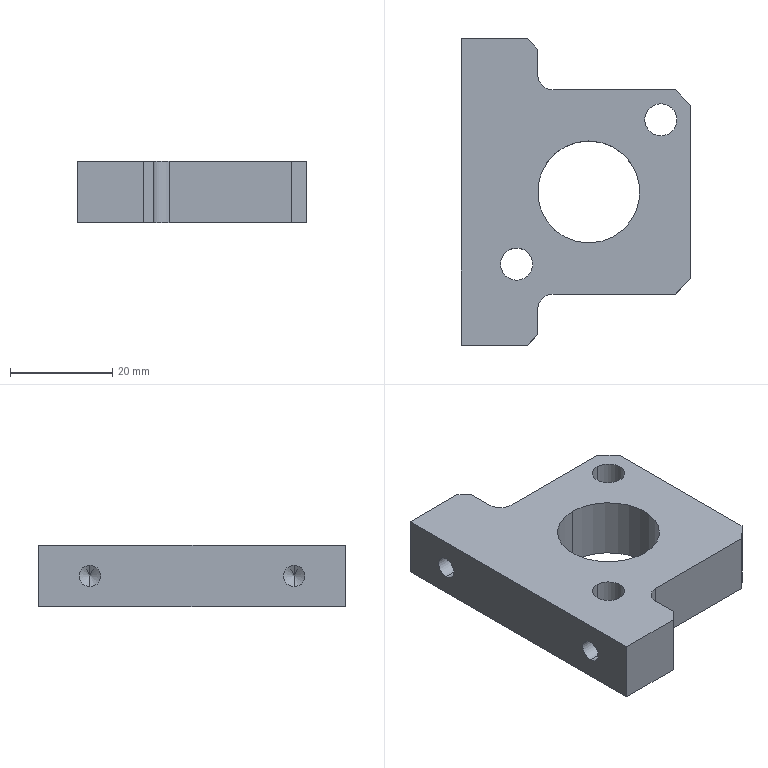Component | SolidWorks | 52-1 | 1 solid | 30 faces | box 45 x 60 x 12 mm | volume 20173 mm3 | plane 14 | cylinder 12 | cone 4 | commonest cylinder face diameters 6.3 x4 4.2 x4 20 x2 6 x2
build123d program:
from build123d import *

# Parameters (mm, degrees)
SKETCH1_R               = 10
BOSS_EXTRUDE1_DEPTH     = 12
FILLET1_R               = 3
M5_TAPPED_HOLE1_D       = 4.2
M5_TAPPED_HOLE1_DEPTH   = 14
M5_TAPPED_HOLE1_TIP     = 1.262
CHAMFER1_SIZE           = 3
SKETCH4_R               = 3.15
CUT_EXTRUDE1_DEPTH      = 12
CIRCULAR_PATTERN1_COUNT = 2
CHAMFER2_SIZE           = 2


with BuildPart() as part:
    # Sketch1 → Boss-Extrude1 (new body)
    with BuildSketch(Plane.XY):
        Polygon((-20, 10), (-30, 10), (-30, 25), (30, 25), (30, 10), (20, 10), (20, -20), (-20, -20), align=None)
        Circle(SKETCH1_R, mode=Mode.SUBTRACT)
    extrude(amount=BOSS_EXTRUDE1_DEPTH)

    # Fillet1
    fillet1_edges = [part.edges().sort_by_distance(p)[0] for p in [
        (20, 10, 6),
        (-20, 10, 6),
    ]]
    fillet(fillet1_edges, radius=FILLET1_R)

    # M5 Tapped Hole1
    with Locations(Plane(origin=(0, 25, 0), x_dir=(1, 0, 0), z_dir=(0, 1, 0))):
        with Locations((-20, -6), (20, -6)):
            Hole(M5_TAPPED_HOLE1_D / 2, depth=M5_TAPPED_HOLE1_DEPTH)
            with Locations((0, 0, -(M5_TAPPED_HOLE1_DEPTH + M5_TAPPED_HOLE1_TIP / 2))):  # 118° drill point
                Cone(0, M5_TAPPED_HOLE1_D / 2, M5_TAPPED_HOLE1_TIP, mode=Mode.SUBTRACT)

    # Chamfer1
    chamfer1_edges = [part.edges().sort_by_distance(p)[0] for p in [
        (20, -20, 6),
        (-20, -20, 6),
    ]]
    chamfer(chamfer1_edges, length=CHAMFER1_SIZE)

    # Sketch4 → Cut-Extrude1 (cut)
    with BuildSketch(Plane.XY.offset(12)):
        with Locations((-14.142, -14.142)):
            Circle(SKETCH4_R)
    cut_extrude1 = extrude(amount=-CUT_EXTRUDE1_DEPTH, mode=Mode.SUBTRACT)

    # Circular Pattern1: Cut-Extrude1 ×2 about axis
    circular_pattern1_axis = Axis((0, 0, 0), (0, 0, 1))
    for i in range(1, CIRCULAR_PATTERN1_COUNT):
        add(cut_extrude1.rotate(circular_pattern1_axis, i * 360 / CIRCULAR_PATTERN1_COUNT), mode=Mode.SUBTRACT)

    # Chamfer2
    chamfer2_edges = [part.edges().sort_by_distance(p)[0] for p in [
        (30, 10, 6),
        (-30, 10, 6),
    ]]
    chamfer(chamfer2_edges, length=CHAMFER2_SIZE)


solid = part.part

# Placed as in the assembly
solid = solid.moved(Location((0, -65.5, 214.893), (180, 0, 90)))
STEP:
#1=CARTESIAN_POINT('',(-0.5568,-3.012,8.46));
#2=VERTEX_POINT('',#1);
#3=CARTESIAN_POINT('',(-0.5568,-3.26,8.46));
#4=VERTEX_POINT('',#3);
#5=CARTESIAN_POINT('',(-0.5568,-3.136,8.46));
#6=DIRECTION('',(0.,-0.,-1.));
#7=DIRECTION('',(0.,1.,0.));
#8=AXIS2_PLACEMENT_3D('',#5,#6,#7);
#9=CIRCLE('',#8,0.124);
#10=EDGE_CURVE('',#2,#4,#9,.T.);
#11=ORIENTED_EDGE('',*,*,#10,.F.);
#12=CARTESIAN_POINT('',(-0.5568,-3.012,7.988));
#13=VERTEX_POINT('',#12);
#14=CARTESIAN_POINT('',(-0.5568,-3.012,8.46));
#15=DIRECTION('',(0.,-0.,-1.));
#16=VECTOR('',#15,39.37);
#17=LINE('',#14,#16);
#18=EDGE_CURVE('',#2,#13,#17,.T.);
#19=ORIENTED_EDGE('',*,*,#18,.T.);
#20=CARTESIAN_POINT('',(-0.5568,-3.26,7.988));
#21=VERTEX_POINT('',#20);
#22=CARTESIAN_POINT('',(-0.5568,-3.136,7.988));
#23=DIRECTION('',(0.,-0.,-1.));
#24=DIRECTION('',(0.,1.,0.));
#25=AXIS2_PLACEMENT_3D('',#22,#23,#24);
#26=CIRCLE('',#25,0.124);
#27=EDGE_CURVE('',#13,#21,#26,.T.);
#28=ORIENTED_EDGE('',*,*,#27,.T.);
#29=CARTESIAN_POINT('',(-0.5568,-3.26,8.46));
#30=DIRECTION('',(0.,-0.,-1.));
#31=VECTOR('',#30,39.37);
#32=LINE('',#29,#31);
#33=EDGE_CURVE('',#4,#21,#32,.T.);
#34=ORIENTED_EDGE('',*,*,#33,.F.);
#35=EDGE_LOOP('',(#11,#19,#28,#34));
#36=FACE_OUTER_BOUND('',#35,.T.);
#37=CARTESIAN_POINT('',(-0.5568,-3.136,8.46));
#38=DIRECTION('',(0.,-0.,-1.));
#39=DIRECTION('',(-0.,-1.,0.));
#40=AXIS2_PLACEMENT_3D('',#37,#38,#39);
#41=CYLINDRICAL_SURFACE('',#40,0.124);
#42=ADVANCED_FACE('',(#36),#41,.F.);
#43=CARTESIAN_POINT('',(0.5568,-1.898,8.46));
#44=VERTEX_POINT('',#43);
#45=CARTESIAN_POINT('',(0.5568,-2.146,8.46));
#46=VERTEX_POINT('',#45);
#47=CARTESIAN_POINT('',(0.5568,-2.022,8.46));
#48=DIRECTION('',(0.,-0.,-1.));
#49=DIRECTION('',(-0.,-1.,0.));
#50=AXIS2_PLACEMENT_3D('',#47,#48,#49);
#51=CIRCLE('',#50,0.124);
#52=EDGE_CURVE('',#44,#46,#51,.T.);
#53=ORIENTED_EDGE('',*,*,#52,.F.);
#54=CARTESIAN_POINT('',(0.5568,-1.898,7.988));
#55=VERTEX_POINT('',#54);
#56=CARTESIAN_POINT('',(0.5568,-1.898,8.46));
#57=DIRECTION('',(0.,-0.,-1.));
#58=VECTOR('',#57,39.37);
#59=LINE('',#56,#58);
#60=EDGE_CURVE('',#44,#55,#59,.T.);
#61=ORIENTED_EDGE('',*,*,#60,.T.);
#62=CARTESIAN_POINT('',(0.5568,-2.146,7.988));
#63=VERTEX_POINT('',#62);
#64=CARTESIAN_POINT('',(0.5568,-2.022,7.988));
#65=DIRECTION('',(0.,-0.,-1.));
#66=DIRECTION('',(-0.,-1.,0.));
#67=AXIS2_PLACEMENT_3D('',#64,#65,#66);
#68=CIRCLE('',#67,0.124);
#69=EDGE_CURVE('',#55,#63,#68,.T.);
#70=ORIENTED_EDGE('',*,*,#69,.T.);
#71=CARTESIAN_POINT('',(0.5568,-2.146,8.46));
#72=DIRECTION('',(0.,-0.,-1.));
#73=VECTOR('',#72,39.37);
#74=LINE('',#71,#73);
#75=EDGE_CURVE('',#46,#63,#74,.T.);
#76=ORIENTED_EDGE('',*,*,#75,.F.);
#77=EDGE_LOOP('',(#53,#61,#70,#76));
#78=FACE_OUTER_BOUND('',#77,.T.);
#79=CARTESIAN_POINT('',(0.5568,-2.022,8.46));
#80=DIRECTION('',(0.,-0.,-1.));
#81=DIRECTION('',(-0.,-1.,0.));
#82=AXIS2_PLACEMENT_3D('',#79,#80,#81);
#83=CYLINDRICAL_SURFACE('',#82,0.124);
#84=ADVANCED_FACE('',(#78),#83,.F.);
#85=CARTESIAN_POINT('',(-0.4331,-1.791,8.307));
#86=VERTEX_POINT('',#85);
#87=CARTESIAN_POINT('',(-0.4331,-1.791,8.141));
#88=VERTEX_POINT('',#87);
#89=CARTESIAN_POINT('',(-0.4331,-1.791,8.224));
#90=DIRECTION('',(-1.,0.,-0.));
#91=DIRECTION('',(0.,0.,-1.));
#92=AXIS2_PLACEMENT_3D('',#89,#90,#91);
#93=CIRCLE('',#92,0.08268);
#94=EDGE_CURVE('',#86,#88,#93,.T.);
#95=ORIENTED_EDGE('',*,*,#94,.F.);
#96=CARTESIAN_POINT('',(-0.9843,-1.791,8.307));
#97=VERTEX_POINT('',#96);
#98=CARTESIAN_POINT('',(-0.9843,-1.791,8.307));
#99=DIRECTION('',(-1.,0.,-0.));
#100=VECTOR('',#99,39.37);
#101=LINE('',#98,#100);
#102=EDGE_CURVE('',#86,#97,#101,.T.);
#103=ORIENTED_EDGE('',*,*,#102,.T.);
#104=CARTESIAN_POINT('',(-0.9843,-1.791,8.141));
#105=VERTEX_POINT('',#104);
#106=CARTESIAN_POINT('',(-0.9843,-1.791,8.224));
#107=DIRECTION('',(-1.,0.,-0.));
#108=DIRECTION('',(0.,0.,-1.));
#109=AXIS2_PLACEMENT_3D('',#106,#107,#108);
#110=CIRCLE('',#109,0.08268);
#111=EDGE_CURVE('',#97,#105,#110,.T.);
#112=ORIENTED_EDGE('',*,*,#111,.T.);
#113=CARTESIAN_POINT('',(-0.9843,-1.791,8.141));
#114=DIRECTION('',(-1.,0.,-0.));
#115=VECTOR('',#114,39.37);
#116=LINE('',#113,#115);
#117=EDGE_CURVE('',#88,#105,#116,.T.);
#118=ORIENTED_EDGE('',*,*,#117,.F.);
#119=EDGE_LOOP('',(#95,#103,#112,#118));
#120=FACE_OUTER_BOUND('',#119,.T.);
#121=CARTESIAN_POINT('',(-0.9843,-1.791,8.224));
#122=DIRECTION('',(-1.,0.,-0.));
#123=DIRECTION('',(0.,0.,-1.));
#124=AXIS2_PLACEMENT_3D('',#121,#122,#123);
#125=CYLINDRICAL_SURFACE('',#124,0.08268);
#126=ADVANCED_FACE('',(#120),#125,.F.);
#127=CARTESIAN_POINT('',(-0.3834,-1.791,8.224));
#128=VERTEX_POINT('',#127);
#129=CARTESIAN_POINT('',(-0.4331,-1.791,8.141));
#130=DIRECTION('',(-0.515,0.,-0.8572));
#131=VECTOR('',#130,39.37);
#132=LINE('',#129,#131);
#133=EDGE_CURVE('',#128,#88,#132,.T.);
#134=ORIENTED_EDGE('',*,*,#133,.F.);
#135=CARTESIAN_POINT('',(-0.4331,-1.791,8.307));
#136=DIRECTION('',(-0.515,0.,0.8572));
#137=VECTOR('',#136,39.37);
#138=LINE('',#135,#137);
#139=EDGE_CURVE('',#128,#86,#138,.T.);
#140=ORIENTED_EDGE('',*,*,#139,.T.);
#141=ORIENTED_EDGE('',*,*,#94,.T.);
#142=EDGE_LOOP('',(#134,#140,#141));
#143=FACE_OUTER_BOUND('',#142,.T.);
#144=CARTESIAN_POINT('',(-0.4331,-1.791,8.224));
#145=DIRECTION('',(-1.,0.,-0.));
#146=DIRECTION('',(0.,0.,-1.));
#147=AXIS2_PLACEMENT_3D('',#144,#145,#146);
#148=CONICAL_SURFACE('',#147,0.08268,1.03);
#149=ADVANCED_FACE('',(#143),#148,.F.);
#150=CARTESIAN_POINT('',(-0.4331,-3.366,8.307));
#151=VERTEX_POINT('',#150);
#152=CARTESIAN_POINT('',(-0.4331,-3.366,8.141));
#153=VERTEX_POINT('',#152);
#154=CARTESIAN_POINT('',(-0.4331,-3.366,8.224));
#155=DIRECTION('',(-1.,0.,-0.));
#156=DIRECTION('',(0.,0.,-1.));
#157=AXIS2_PLACEMENT_3D('',#154,#155,#156);
#158=CIRCLE('',#157,0.08268);
#159=EDGE_CURVE('',#151,#153,#158,.T.);
#160=ORIENTED_EDGE('',*,*,#159,.F.);
#161=CARTESIAN_POINT('',(-0.9843,-3.366,8.307));
#162=VERTEX_POINT('',#161);
#163=CARTESIAN_POINT('',(-0.9843,-3.366,8.307));
#164=DIRECTION('',(-1.,0.,-0.));
#165=VECTOR('',#164,39.37);
#166=LINE('',#163,#165);
#167=EDGE_CURVE('',#151,#162,#166,.T.);
#168=ORIENTED_EDGE('',*,*,#167,.T.);
#169=CARTESIAN_POINT('',(-0.9843,-3.366,8.141));
#170=VERTEX_POINT('',#169);
#171=CARTESIAN_POINT('',(-0.9843,-3.366,8.224));
#172=DIRECTION('',(-1.,0.,-0.));
#173=DIRECTION('',(0.,0.,-1.));
#174=AXIS2_PLACEMENT_3D('',#171,#172,#173);
#175=CIRCLE('',#174,0.08268);
#176=EDGE_CURVE('',#162,#170,#175,.T.);
#177=ORIENTED_EDGE('',*,*,#176,.T.);
#178=CARTESIAN_POINT('',(-0.9843,-3.366,8.141));
#179=DIRECTION('',(-1.,0.,-0.));
#180=VECTOR('',#179,39.37);
#181=LINE('',#178,#180);
#182=EDGE_CURVE('',#153,#170,#181,.T.);
#183=ORIENTED_EDGE('',*,*,#182,.F.);
#184=EDGE_LOOP('',(#160,#168,#177,#183));
#185=FACE_OUTER_BOUND('',#184,.T.);
#186=CARTESIAN_POINT('',(-0.9843,-3.366,8.224));
#187=DIRECTION('',(-1.,0.,-0.));
#188=DIRECTION('',(0.,0.,-1.));
#189=AXIS2_PLACEMENT_3D('',#186,#187,#188);
#190=CYLINDRICAL_SURFACE('',#189,0.08268);
#191=ADVANCED_FACE('',(#185),#190,.F.);
#192=CARTESIAN_POINT('',(-0.3834,-3.366,8.224));
#193=VERTEX_POINT('',#192);
#194=CARTESIAN_POINT('',(-0.4331,-3.366,8.141));
#195=DIRECTION('',(-0.515,0.,-0.8572));
#196=VECTOR('',#195,39.37);
#197=LINE('',#194,#196);
#198=EDGE_CURVE('',#193,#153,#197,.T.);
#199=ORIENTED_EDGE('',*,*,#198,.F.);
#200=CARTESIAN_POINT('',(-0.4331,-3.366,8.307));
#201=DIRECTION('',(-0.515,0.,0.8572));
#202=VECTOR('',#201,39.37);
#203=LINE('',#200,#202);
#204=EDGE_CURVE('',#193,#151,#203,.T.);
#205=ORIENTED_EDGE('',*,*,#204,.T.);
#206=ORIENTED_EDGE('',*,*,#159,.T.);
#207=EDGE_LOOP('',(#199,#205,#206));
#208=FACE_OUTER_BOUND('',#207,.T.);
#209=CARTESIAN_POINT('',(-0.4331,-3.366,8.224));
#210=DIRECTION('',(-1.,0.,-0.));
#211=DIRECTION('',(0.,0.,-1.));
#212=AXIS2_PLACEMENT_3D('',#209,#210,#211);
#213=CONICAL_SURFACE('',#212,0.08268,1.03);
#214=ADVANCED_FACE('',(#208),#213,.F.);
#215=CARTESIAN_POINT('',(-0.,-2.185,7.988));
#216=VERTEX_POINT('',#215);
#217=CARTESIAN_POINT('',(-0.,-2.972,7.988));
#218=VERTEX_POINT('',#217);
#219=CARTESIAN_POINT('',(-0.,-2.579,7.988));
#220=DIRECTION('',(0.,-0.,-1.));
#221=DIRECTION('',(-0.,-1.,0.));
#222=AXIS2_PLACEMENT_3D('',#219,#220,#221);
#223=CIRCLE('',#222,0.3937);
#224=EDGE_CURVE('',#216,#218,#223,.T.);
#225=ORIENTED_EDGE('',*,*,#224,.T.);
#226=CARTESIAN_POINT('',(-0.,-2.972,8.46));
#227=VERTEX_POINT('',#226);
#228=CARTESIAN_POINT('',(-0.,-2.972,7.988));
#229=DIRECTION('',(-0.,0.,1.));
#230=VECTOR('',#229,39.37);
#231=LINE('',#228,#230);
#232=EDGE_CURVE('',#218,#227,#231,.T.);
#233=ORIENTED_EDGE('',*,*,#232,.T.);
#234=CARTESIAN_POINT('',(-0.,-2.185,8.46));
#235=VERTEX_POINT('',#234);
#236=CARTESIAN_POINT('',(-0.,-2.579,8.46));
#237=DIRECTION('',(0.,-0.,-1.));
#238=DIRECTION('',(-0.,-1.,0.));
#239=AXIS2_PLACEMENT_3D('',#236,#237,#238);
#240=CIRCLE('',#239,0.3937);
#241=EDGE_CURVE('',#235,#227,#240,.T.);
#242=ORIENTED_EDGE('',*,*,#241,.F.);
#243=CARTESIAN_POINT('',(-0.,-2.185,7.988));
#244=DIRECTION('',(-0.,0.,1.));
#245=VECTOR('',#244,39.37);
#246=LINE('',#243,#245);
#247=EDGE_CURVE('',#216,#235,#246,.T.);
#248=ORIENTED_EDGE('',*,*,#247,.F.);
#249=EDGE_LOOP('',(#225,#233,#242,#248));
#250=FACE_OUTER_BOUND('',#249,.T.);
#251=CARTESIAN_POINT('',(-0.,-2.579,7.988));
#252=DIRECTION('',(-0.,0.,1.));
#253=DIRECTION('',(0.,1.,0.));
#254=AXIS2_PLACEMENT_3D('',#251,#252,#253);
#255=CYLINDRICAL_SURFACE('',#254,0.3937);
#256=ADVANCED_FACE('',(#250),#255,.F.);
#257=CARTESIAN_POINT('',(-0.5568,-3.136,7.988));
#258=DIRECTION('',(0.,-0.,-1.));
#259=DIRECTION('',(0.,1.,0.));
#260=AXIS2_PLACEMENT_3D('',#257,#258,#259);
#261=CIRCLE('',#260,0.124);
#262=EDGE_CURVE('',#21,#13,#261,.T.);
#263=ORIENTED_EDGE('',*,*,#262,.F.);
#264=ORIENTED_EDGE('',*,*,#27,.F.);
#265=EDGE_LOOP('',(#263,#264));
#266=FACE_BOUND('',#265,.T.);
#267=CARTESIAN_POINT('',(0.5568,-2.022,7.988));
#268=DIRECTION('',(0.,-0.,-1.));
#269=DIRECTION('',(-0.,-1.,0.));
#270=AXIS2_PLACEMENT_3D('',#267,#268,#269);
#271=CIRCLE('',#270,0.124);
#272=EDGE_CURVE('',#63,#55,#271,.T.);
#273=ORIENTED_EDGE('',*,*,#272,.F.);
#274=ORIENTED_EDGE('',*,*,#69,.F.);
#275=EDGE_LOOP('',(#273,#274));
#276=FACE_BOUND('',#275,.T.);
#277=CARTESIAN_POINT('',(-0.3937,-3.484,7.988));
#278=VERTEX_POINT('',#277);
#279=CARTESIAN_POINT('',(-0.3937,-3.681,7.988));
#280=VERTEX_POINT('',#279);
#281=CARTESIAN_POINT('',(-0.3937,-3.366,7.988));
#282=DIRECTION('',(-0.,-1.,0.));
#283=VECTOR('',#282,39.37);
#284=LINE('',#281,#283);
#285=EDGE_CURVE('',#278,#280,#284,.T.);
#286=ORIENTED_EDGE('',*,*,#285,.T.);
#287=CARTESIAN_POINT('',(-0.4724,-3.76,7.988));
#288=VERTEX_POINT('',#287);
#289=CARTESIAN_POINT('',(-0.4724,-3.76,7.988));
#290=DIRECTION('',(-0.7071,-0.7071,0.));
#291=VECTOR('',#290,39.37);
#292=LINE('',#289,#291);
#293=EDGE_CURVE('',#280,#288,#292,.T.);
#294=ORIENTED_EDGE('',*,*,#293,.T.);
#295=CARTESIAN_POINT('',(-0.9843,-3.76,7.988));
#296=VERTEX_POINT('',#295);
#297=CARTESIAN_POINT('',(-0.3937,-3.76,7.988));
#298=DIRECTION('',(-1.,0.,-0.));
#299=VECTOR('',#298,39.37);
#300=LINE('',#297,#299);
#301=EDGE_CURVE('',#288,#296,#300,.T.);
#302=ORIENTED_EDGE('',*,*,#301,.T.);
#303=CARTESIAN_POINT('',(-0.9843,-1.398,7.988));
#304=VERTEX_POINT('',#303);
#305=CARTESIAN_POINT('',(-0.9843,-1.398,7.988));
#306=DIRECTION('',(0.,1.,-0.));
#307=VECTOR('',#306,39.37);
#308=LINE('',#305,#307);
#309=EDGE_CURVE('',#296,#304,#308,.T.);
#310=ORIENTED_EDGE('',*,*,#309,.T.);
#311=CARTESIAN_POINT('',(-0.4724,-1.398,7.988));
#312=VERTEX_POINT('',#311);
#313=CARTESIAN_POINT('',(-0.3937,-1.398,7.988));
#314=DIRECTION('',(1.,-0.,0.));
#315=VECTOR('',#314,39.37);
#316=LINE('',#313,#315);
#317=EDGE_CURVE('',#304,#312,#316,.T.);
#318=ORIENTED_EDGE('',*,*,#317,.T.);
#319=CARTESIAN_POINT('',(-0.3937,-1.476,7.988));
#320=VERTEX_POINT('',#319);
#321=CARTESIAN_POINT('',(-0.3937,-1.476,7.988));
#322=DIRECTION('',(0.7071,-0.7071,0.));
#323=VECTOR('',#322,39.37);
#324=LINE('',#321,#323);
#325=EDGE_CURVE('',#312,#320,#324,.T.);
#326=ORIENTED_EDGE('',*,*,#325,.T.);
#327=CARTESIAN_POINT('',(-0.3937,-1.673,7.988));
#328=VERTEX_POINT('',#327);
#329=CARTESIAN_POINT('',(-0.3937,-1.791,7.988));
#330=DIRECTION('',(-0.,-1.,0.));
#331=VECTOR('',#330,39.37);
#332=LINE('',#329,#331);
#333=EDGE_CURVE('',#320,#328,#332,.T.);
#334=ORIENTED_EDGE('',*,*,#333,.T.);
#335=CARTESIAN_POINT('',(-0.2756,-1.791,7.988));
#336=VERTEX_POINT('',#335);
#337=CARTESIAN_POINT('',(-0.2756,-1.673,7.988));
#338=DIRECTION('',(-0.,0.,1.));
#339=DIRECTION('',(0.,1.,0.));
#340=AXIS2_PLACEMENT_3D('',#337,#338,#339);
#341=CIRCLE('',#340,0.1181);
#342=EDGE_CURVE('',#328,#336,#341,.T.);
#343=ORIENTED_EDGE('',*,*,#342,.T.);
#344=CARTESIAN_POINT('',(0.6693,-1.791,7.988));
#345=VERTEX_POINT('',#344);
#346=CARTESIAN_POINT('',(-0.3937,-1.791,7.988));
#347=DIRECTION('',(1.,-0.,0.));
#348=VECTOR('',#347,39.37);
#349=LINE('',#346,#348);
#350=EDGE_CURVE('',#336,#345,#349,.T.);
#351=ORIENTED_EDGE('',*,*,#350,.T.);
#352=CARTESIAN_POINT('',(0.7874,-1.909,7.988));
#353=VERTEX_POINT('',#352);
#354=CARTESIAN_POINT('',(0.7874,-1.909,7.988));
#355=DIRECTION('',(0.7071,-0.7071,0.));
#356=VECTOR('',#355,39.37);
#357=LINE('',#354,#356);
#358=EDGE_CURVE('',#345,#353,#357,.T.);
#359=ORIENTED_EDGE('',*,*,#358,.T.);
#360=CARTESIAN_POINT('',(0.7874,-3.248,7.988));
#361=VERTEX_POINT('',#360);
#362=CARTESIAN_POINT('',(0.7874,-1.791,7.988));
#363=DIRECTION('',(-0.,-1.,0.));
#364=VECTOR('',#363,39.37);
#365=LINE('',#362,#364);
#366=EDGE_CURVE('',#353,#361,#365,.T.);
#367=ORIENTED_EDGE('',*,*,#366,.T.);
#368=CARTESIAN_POINT('',(0.6693,-3.366,7.988));
#369=VERTEX_POINT('',#368);
#370=CARTESIAN_POINT('',(0.6693,-3.366,7.988));
#371=DIRECTION('',(-0.7071,-0.7071,0.));
#372=VECTOR('',#371,39.37);
#373=LINE('',#370,#372);
#374=EDGE_CURVE('',#361,#369,#373,.T.);
#375=ORIENTED_EDGE('',*,*,#374,.T.);
#376=CARTESIAN_POINT('',(-0.2756,-3.366,7.988));
#377=VERTEX_POINT('',#376);
#378=CARTESIAN_POINT('',(-0.3937,-3.366,7.988));
#379=DIRECTION('',(-1.,0.,-0.));
#380=VECTOR('',#379,39.37);
#381=LINE('',#378,#380);
#382=EDGE_CURVE('',#369,#377,#381,.T.);
#383=ORIENTED_EDGE('',*,*,#382,.T.);
#384=CARTESIAN_POINT('',(-0.2756,-3.484,7.988));
#385=DIRECTION('',(-0.,0.,1.));
#386=DIRECTION('',(0.,1.,0.));
#387=AXIS2_PLACEMENT_3D('',#384,#385,#386);
#388=CIRCLE('',#387,0.1181);
#389=EDGE_CURVE('',#377,#278,#388,.T.);
#390=ORIENTED_EDGE('',*,*,#389,.T.);
#391=EDGE_LOOP('',(#286,#294,#302,#310,#318,#326,#334,#343,#351,#359,#367,#375,#383,#390));
#392=FACE_OUTER_BOUND('',#391,.T.);
#393=ORIENTED_EDGE('',*,*,#224,.F.);
#394=CARTESIAN_POINT('',(-0.,-2.579,7.988));
#395=DIRECTION('',(0.,-0.,-1.));
#396=DIRECTION('',(-0.,-1.,0.));
#397=AXIS2_PLACEMENT_3D('',#394,#395,#396);
#398=CIRCLE('',#397,0.3937);
#399=EDGE_CURVE('',#218,#216,#398,.T.);
#400=ORIENTED_EDGE('',*,*,#399,.F.);
#401=EDGE_LOOP('',(#393,#400));
#402=FACE_BOUND('',#401,.T.);
#403=CARTESIAN_POINT('',(-0.,-2.579,7.988));
#404=DIRECTION('',(-0.,0.,1.));
#405=DIRECTION('',(0.,1.,-0.));
#406=AXIS2_PLACEMENT_3D('',#403,#404,#405);
#407=PLANE('',#406);
#408=ADVANCED_FACE('',(#266,#276,#392,#402),#407,.F.);
#409=CARTESIAN_POINT('',(-0.5568,-3.136,8.46));
#410=DIRECTION('',(0.,-0.,-1.));
#411=DIRECTION('',(0.,1.,0.));
#412=AXIS2_PLACEMENT_3D('',#409,#410,#411);
#413=CIRCLE('',#412,0.124);
#414=EDGE_CURVE('',#4,#2,#413,.T.);
#415=ORIENTED_EDGE('',*,*,#414,.T.);
#416=ORIENTED_EDGE('',*,*,#10,.T.);
#417=EDGE_LOOP('',(#415,#416));
#418=FACE_BOUND('',#417,.T.);
#419=CARTESIAN_POINT('',(0.5568,-2.022,8.46));
#420=DIRECTION('',(0.,-0.,-1.));
#421=DIRECTION('',(-0.,-1.,0.));
#422=AXIS2_PLACEMENT_3D('',#419,#420,#421);
#423=CIRCLE('',#422,0.124);
#424=EDGE_CURVE('',#46,#44,#423,.T.);
#425=ORIENTED_EDGE('',*,*,#424,.T.);
#426=ORIENTED_EDGE('',*,*,#52,.T.);
#427=EDGE_LOOP('',(#425,#426));
#428=FACE_BOUND('',#427,.T.);
#429=CARTESIAN_POINT('',(-0.4724,-3.76,8.46));
#430=VERTEX_POINT('',#429);
#431=CARTESIAN_POINT('',(-0.9843,-3.76,8.46));
#432=VERTEX_POINT('',#431);
#433=CARTESIAN_POINT('',(-0.3937,-3.76,8.46));
#434=DIRECTION('',(-1.,0.,-0.));
#435=VECTOR('',#434,39.37);
#436=LINE('',#433,#435);
#437=EDGE_CURVE('',#430,#432,#436,.T.);
#438=ORIENTED_EDGE('',*,*,#437,.F.);
#439=CARTESIAN_POINT('',(-0.3937,-3.681,8.46));
#440=VERTEX_POINT('',#439);
#441=CARTESIAN_POINT('',(0.3543,-2.933,8.46));
#442=DIRECTION('',(0.7071,0.7071,-0.));
#443=VECTOR('',#442,39.37);
#444=LINE('',#441,#443);
#445=EDGE_CURVE('',#430,#440,#444,.T.);
#446=ORIENTED_EDGE('',*,*,#445,.T.);
#447=CARTESIAN_POINT('',(-0.3937,-3.484,8.46));
#448=VERTEX_POINT('',#447);
#449=CARTESIAN_POINT('',(-0.3937,-3.366,8.46));
#450=DIRECTION('',(-0.,-1.,0.));
#451=VECTOR('',#450,39.37);
#452=LINE('',#449,#451);
#453=EDGE_CURVE('',#448,#440,#452,.T.);
#454=ORIENTED_EDGE('',*,*,#453,.F.);
#455=CARTESIAN_POINT('',(-0.2756,-3.366,8.46));
#456=VERTEX_POINT('',#455);
#457=CARTESIAN_POINT('',(-0.2756,-3.484,8.46));
#458=DIRECTION('',(0.,-0.,-1.));
#459=DIRECTION('',(0.,1.,0.));
#460=AXIS2_PLACEMENT_3D('',#457,#458,#459);
#461=CIRCLE('',#460,0.1181);
#462=EDGE_CURVE('',#448,#456,#461,.T.);
#463=ORIENTED_EDGE('',*,*,#462,.T.);
#464=CARTESIAN_POINT('',(0.6693,-3.366,8.46));
#465=VERTEX_POINT('',#464);
#466=CARTESIAN_POINT('',(-0.3937,-3.366,8.46));
#467=DIRECTION('',(-1.,0.,-0.));
#468=VECTOR('',#467,39.37);
#469=LINE('',#466,#468);
#470=EDGE_CURVE('',#465,#456,#469,.T.);
#471=ORIENTED_EDGE('',*,*,#470,.F.);
#472=CARTESIAN_POINT('',(0.7874,-3.248,8.46));
#473=VERTEX_POINT('',#472);
#474=CARTESIAN_POINT('',(0.7283,-3.307,8.46));
#475=DIRECTION('',(0.7071,0.7071,-0.));
#476=VECTOR('',#475,39.37);
#477=LINE('',#474,#476);
#478=EDGE_CURVE('',#465,#473,#477,.T.);
#479=ORIENTED_EDGE('',*,*,#478,.T.);
#480=CARTESIAN_POINT('',(0.7874,-1.909,8.46));
#481=VERTEX_POINT('',#480);
#482=CARTESIAN_POINT('',(0.7874,-1.791,8.46));
#483=DIRECTION('',(-0.,-1.,0.));
#484=VECTOR('',#483,39.37);
#485=LINE('',#482,#484);
#486=EDGE_CURVE('',#481,#473,#485,.T.);
#487=ORIENTED_EDGE('',*,*,#486,.F.);
#488=CARTESIAN_POINT('',(0.6693,-1.791,8.46));
#489=VERTEX_POINT('',#488);
#490=CARTESIAN_POINT('',(0.7283,-1.85,8.46));
#491=DIRECTION('',(-0.7071,0.7071,-0.));
#492=VECTOR('',#491,39.37);
#493=LINE('',#490,#492);
#494=EDGE_CURVE('',#481,#489,#493,.T.);
#495=ORIENTED_EDGE('',*,*,#494,.T.);
#496=CARTESIAN_POINT('',(-0.2756,-1.791,8.46));
#497=VERTEX_POINT('',#496);
#498=CARTESIAN_POINT('',(-0.3937,-1.791,8.46));
#499=DIRECTION('',(1.,-0.,0.));
#500=VECTOR('',#499,39.37);
#501=LINE('',#498,#500);
#502=EDGE_CURVE('',#497,#489,#501,.T.);
#503=ORIENTED_EDGE('',*,*,#502,.F.);
#504=CARTESIAN_POINT('',(-0.3937,-1.673,8.46));
#505=VERTEX_POINT('',#504);
#506=CARTESIAN_POINT('',(-0.2756,-1.673,8.46));
#507=DIRECTION('',(0.,-0.,-1.));
#508=DIRECTION('',(0.,1.,0.));
#509=AXIS2_PLACEMENT_3D('',#506,#507,#508);
#510=CIRCLE('',#509,0.1181);
#511=EDGE_CURVE('',#497,#505,#510,.T.);
#512=ORIENTED_EDGE('',*,*,#511,.T.);
#513=CARTESIAN_POINT('',(-0.3937,-1.476,8.46));
#514=VERTEX_POINT('',#513);
#515=CARTESIAN_POINT('',(-0.3937,-1.791,8.46));
#516=DIRECTION('',(-0.,-1.,0.));
#517=VECTOR('',#516,39.37);
#518=LINE('',#515,#517);
#519=EDGE_CURVE('',#514,#505,#518,.T.);
#520=ORIENTED_EDGE('',*,*,#519,.F.);
#521=CARTESIAN_POINT('',(-0.4724,-1.398,8.46));
#522=VERTEX_POINT('',#521);
#523=CARTESIAN_POINT('',(0.3543,-2.224,8.46));
#524=DIRECTION('',(-0.7071,0.7071,-0.));
#525=VECTOR('',#524,39.37);
#526=LINE('',#523,#525);
#527=EDGE_CURVE('',#514,#522,#526,.T.);
#528=ORIENTED_EDGE('',*,*,#527,.T.);
#529=CARTESIAN_POINT('',(-0.9843,-1.398,8.46));
#530=VERTEX_POINT('',#529);
#531=CARTESIAN_POINT('',(-0.3937,-1.398,8.46));
#532=DIRECTION('',(1.,-0.,0.));
#533=VECTOR('',#532,39.37);
#534=LINE('',#531,#533);
#535=EDGE_CURVE('',#530,#522,#534,.T.);
#536=ORIENTED_EDGE('',*,*,#535,.F.);
#537=CARTESIAN_POINT('',(-0.9843,-1.398,8.46));
#538=DIRECTION('',(0.,1.,-0.));
#539=VECTOR('',#538,39.37);
#540=LINE('',#537,#539);
#541=EDGE_CURVE('',#432,#530,#540,.T.);
#542=ORIENTED_EDGE('',*,*,#541,.F.);
#543=EDGE_LOOP('',(#438,#446,#454,#463,#471,#479,#487,#495,#503,#512,#520,#528,#536,#542));
#544=FACE_OUTER_BOUND('',#543,.T.);
#545=ORIENTED_EDGE('',*,*,#241,.T.);
#546=CARTESIAN_POINT('',(-0.,-2.579,8.46));
#547=DIRECTION('',(0.,-0.,-1.));
#548=DIRECTION('',(-0.,-1.,0.));
#549=AXIS2_PLACEMENT_3D('',#546,#547,#548);
#550=CIRCLE('',#549,0.3937);
#551=EDGE_CURVE('',#227,#235,#550,.T.);
#552=ORIENTED_EDGE('',*,*,#551,.T.);
#553=EDGE_LOOP('',(#545,#552));
#554=FACE_BOUND('',#553,.T.);
#555=CARTESIAN_POINT('',(-0.,-2.579,8.46));
#556=DIRECTION('',(-0.,0.,1.));
#557=DIRECTION('',(0.,1.,-0.));
#558=AXIS2_PLACEMENT_3D('',#555,#556,#557);
#559=PLANE('',#558);
#560=ADVANCED_FACE('',(#418,#428,#544,#554),#559,.T.);
#561=ORIENTED_EDGE('',*,*,#301,.F.);
#562=CARTESIAN_POINT('',(-0.4724,-3.76,7.988));
#563=DIRECTION('',(-0.,0.,1.));
#564=VECTOR('',#563,39.37);
#565=LINE('',#562,#564);
#566=EDGE_CURVE('',#288,#430,#565,.T.);
#567=ORIENTED_EDGE('',*,*,#566,.T.);
#568=ORIENTED_EDGE('',*,*,#437,.T.);
#569=CARTESIAN_POINT('',(-0.9843,-3.76,7.988));
#570=DIRECTION('',(-0.,0.,1.));
#571=VECTOR('',#570,39.37);
#572=LINE('',#569,#571);
#573=EDGE_CURVE('',#296,#432,#572,.T.);
#574=ORIENTED_EDGE('',*,*,#573,.F.);
#575=EDGE_LOOP('',(#561,#567,#568,#574));
#576=FACE_OUTER_BOUND('',#575,.T.);
#577=CARTESIAN_POINT('',(-0.3937,-3.76,7.988));
#578=DIRECTION('',(0.,1.,-0.));
#579=DIRECTION('',(0.,-0.,-1.));
#580=AXIS2_PLACEMENT_3D('',#577,#578,#579);
#581=PLANE('',#580);
#582=ADVANCED_FACE('',(#576),#581,.F.);
#583=CARTESIAN_POINT('',(-0.9843,-1.791,8.224));
#584=DIRECTION('',(-1.,0.,-0.));
#585=DIRECTION('',(0.,0.,-1.));
#586=AXIS2_PLACEMENT_3D('',#583,#584,#585);
#587=CIRCLE('',#586,0.08268);
#588=EDGE_CURVE('',#105,#97,#587,.T.);
#589=ORIENTED_EDGE('',*,*,#588,.F.);
#590=ORIENTED_EDGE('',*,*,#111,.F.);
#591=EDGE_LOOP('',(#589,#590));
#592=FACE_BOUND('',#591,.T.);
#593=CARTESIAN_POINT('',(-0.9843,-3.366,8.224));
#594=DIRECTION('',(-1.,0.,-0.));
#595=DIRECTION('',(0.,0.,-1.));
#596=AXIS2_PLACEMENT_3D('',#593,#594,#595);
#597=CIRCLE('',#596,0.08268);
#598=EDGE_CURVE('',#170,#162,#597,.T.);
#599=ORIENTED_EDGE('',*,*,#598,.F.);
#600=ORIENTED_EDGE('',*,*,#176,.F.);
#601=EDGE_LOOP('',(#599,#600));
#602=FACE_BOUND('',#601,.T.);
#603=ORIENTED_EDGE('',*,*,#541,.T.);
#604=CARTESIAN_POINT('',(-0.9843,-1.398,7.988));
#605=DIRECTION('',(-0.,0.,1.));
#606=VECTOR('',#605,39.37);
#607=LINE('',#604,#606);
#608=EDGE_CURVE('',#304,#530,#607,.T.);
#609=ORIENTED_EDGE('',*,*,#608,.F.);
#610=ORIENTED_EDGE('',*,*,#309,.F.);
#611=ORIENTED_EDGE('',*,*,#573,.T.);
#612=EDGE_LOOP('',(#603,#609,#610,#611));
#613=FACE_OUTER_BOUND('',#612,.T.);
#614=CARTESIAN_POINT('',(-0.9843,-1.398,7.988));
#615=DIRECTION('',(1.,-0.,0.));
#616=DIRECTION('',(-0.,0.,1.));
#617=AXIS2_PLACEMENT_3D('',#614,#615,#616);
#618=PLANE('',#617);
#619=ADVANCED_FACE('',(#592,#602,#613),#618,.F.);
#620=ORIENTED_EDGE('',*,*,#535,.T.);
#621=CARTESIAN_POINT('',(-0.4724,-1.398,7.988));
#622=DIRECTION('',(0.,-0.,-1.));
#623=VECTOR('',#622,39.37);
#624=LINE('',#621,#623);
#625=EDGE_CURVE('',#522,#312,#624,.T.);
#626=ORIENTED_EDGE('',*,*,#625,.T.);
#627=ORIENTED_EDGE('',*,*,#317,.F.);
#628=ORIENTED_EDGE('',*,*,#608,.T.);
#629=EDGE_LOOP('',(#620,#626,#627,#628));
#630=FACE_OUTER_BOUND('',#629,.T.);
#631=CARTESIAN_POINT('',(-0.3937,-1.398,7.988));
#632=DIRECTION('',(-0.,-1.,0.));
#633=DIRECTION('',(-0.,0.,1.));
#634=AXIS2_PLACEMENT_3D('',#631,#632,#633);
#635=PLANE('',#634);
#636=ADVANCED_FACE('',(#630),#635,.F.);
#637=ORIENTED_EDGE('',*,*,#333,.F.);
#638=CARTESIAN_POINT('',(-0.3937,-1.476,7.988));
#639=DIRECTION('',(-0.,0.,1.));
#640=VECTOR('',#639,39.37);
#641=LINE('',#638,#640);
#642=EDGE_CURVE('',#320,#514,#641,.T.);
#643=ORIENTED_EDGE('',*,*,#642,.T.);
#644=ORIENTED_EDGE('',*,*,#519,.T.);
#645=CARTESIAN_POINT('',(-0.3937,-1.673,7.988));
#646=DIRECTION('',(0.,-0.,-1.));
#647=VECTOR('',#646,39.37);
#648=LINE('',#645,#647);
#649=EDGE_CURVE('',#505,#328,#648,.T.);
#650=ORIENTED_EDGE('',*,*,#649,.T.);
#651=EDGE_LOOP('',(#637,#643,#644,#650));
#652=FACE_OUTER_BOUND('',#651,.T.);
#653=CARTESIAN_POINT('',(-0.3937,-1.791,7.988));
#654=DIRECTION('',(-1.,0.,-0.));
#655=DIRECTION('',(0.,1.,-0.));
#656=AXIS2_PLACEMENT_3D('',#653,#654,#655);
#657=PLANE('',#656);
#658=ADVANCED_FACE('',(#652),#657,.F.);
#659=ORIENTED_EDGE('',*,*,#502,.T.);
#660=CARTESIAN_POINT('',(0.6693,-1.791,7.988));
#661=DIRECTION('',(0.,-0.,-1.));
#662=VECTOR('',#661,39.37);
#663=LINE('',#660,#662);
#664=EDGE_CURVE('',#489,#345,#663,.T.);
#665=ORIENTED_EDGE('',*,*,#664,.T.);
#666=ORIENTED_EDGE('',*,*,#350,.F.);
#667=CARTESIAN_POINT('',(-0.2756,-1.791,8.46));
#668=DIRECTION('',(-0.,0.,1.));
#669=VECTOR('',#668,39.37);
#670=LINE('',#667,#669);
#671=EDGE_CURVE('',#336,#497,#670,.T.);
#672=ORIENTED_EDGE('',*,*,#671,.T.);
#673=EDGE_LOOP('',(#659,#665,#666,#672));
#674=FACE_OUTER_BOUND('',#673,.T.);
#675=CARTESIAN_POINT('',(-0.3937,-1.791,7.988));
#676=DIRECTION('',(-0.,-1.,0.));
#677=DIRECTION('',(-0.,0.,1.));
#678=AXIS2_PLACEMENT_3D('',#675,#676,#677);
#679=PLANE('',#678);
#680=ADVANCED_FACE('',(#674),#679,.F.);
#681=ORIENTED_EDGE('',*,*,#486,.T.);
#682=CARTESIAN_POINT('',(0.7874,-3.248,7.988));
#683=DIRECTION('',(0.,-0.,-1.));
#684=VECTOR('',#683,39.37);
#685=LINE('',#682,#684);
#686=EDGE_CURVE('',#473,#361,#685,.T.);
#687=ORIENTED_EDGE('',*,*,#686,.T.);
#688=ORIENTED_EDGE('',*,*,#366,.F.);
#689=CARTESIAN_POINT('',(0.7874,-1.909,7.988));
#690=DIRECTION('',(-0.,0.,1.));
#691=VECTOR('',#690,39.37);
#692=LINE('',#689,#691);
#693=EDGE_CURVE('',#353,#481,#692,.T.);
#694=ORIENTED_EDGE('',*,*,#693,.T.);
#695=EDGE_LOOP('',(#681,#687,#688,#694));
#696=FACE_OUTER_BOUND('',#695,.T.);
#697=CARTESIAN_POINT('',(0.7874,-1.791,7.988));
#698=DIRECTION('',(-1.,0.,-0.));
#699=DIRECTION('',(0.,-0.,-1.));
#700=AXIS2_PLACEMENT_3D('',#697,#698,#699);
#701=PLANE('',#700);
#702=ADVANCED_FACE('',(#696),#701,.F.);
#703=ORIENTED_EDGE('',*,*,#382,.F.);
#704=CARTESIAN_POINT('',(0.6693,-3.366,7.988));
#705=DIRECTION('',(-0.,0.,1.));
#706=VECTOR('',#705,39.37);
#707=LINE('',#704,#706);
#708=EDGE_CURVE('',#369,#465,#707,.T.);
#709=ORIENTED_EDGE('',*,*,#708,.T.);
#710=ORIENTED_EDGE('',*,*,#470,.T.);
#711=CARTESIAN_POINT('',(-0.2756,-3.366,7.988));
#712=DIRECTION('',(0.,-0.,-1.));
#713=VECTOR('',#712,39.37);
#714=LINE('',#711,#713);
#715=EDGE_CURVE('',#456,#377,#714,.T.);
#716=ORIENTED_EDGE('',*,*,#715,.T.);
#717=EDGE_LOOP('',(#703,#709,#710,#716));
#718=FACE_OUTER_BOUND('',#717,.T.);
#719=CARTESIAN_POINT('',(-0.3937,-3.366,7.988));
#720=DIRECTION('',(0.,1.,-0.));
#721=DIRECTION('',(1.,-0.,0.));
#722=AXIS2_PLACEMENT_3D('',#719,#720,#721);
#723=PLANE('',#722);
#724=ADVANCED_FACE('',(#718),#723,.F.);
#725=ORIENTED_EDGE('',*,*,#453,.T.);
#726=CARTESIAN_POINT('',(-0.3937,-3.681,7.988));
#727=DIRECTION('',(0.,-0.,-1.));
#728=VECTOR('',#727,39.37);
#729=LINE('',#726,#728);
#730=EDGE_CURVE('',#440,#280,#729,.T.);
#731=ORIENTED_EDGE('',*,*,#730,.T.);
#732=ORIENTED_EDGE('',*,*,#285,.F.);
#733=CARTESIAN_POINT('',(-0.3937,-3.484,8.46));
#734=DIRECTION('',(-0.,0.,1.));
#735=VECTOR('',#734,39.37);
#736=LINE('',#733,#735);
#737=EDGE_CURVE('',#278,#448,#736,.T.);
#738=ORIENTED_EDGE('',*,*,#737,.T.);
#739=EDGE_LOOP('',(#725,#731,#732,#738));
#740=FACE_OUTER_BOUND('',#739,.T.);
#741=CARTESIAN_POINT('',(-0.3937,-3.366,7.988));
#742=DIRECTION('',(-1.,0.,-0.));
#743=DIRECTION('',(0.,1.,-0.));
#744=AXIS2_PLACEMENT_3D('',#741,#742,#743);
#745=PLANE('',#744);
#746=ADVANCED_FACE('',(#740),#745,.F.);
#747=ORIENTED_EDGE('',*,*,#232,.F.);
#748=ORIENTED_EDGE('',*,*,#399,.T.);
#749=ORIENTED_EDGE('',*,*,#247,.T.);
#750=ORIENTED_EDGE('',*,*,#551,.F.);
#751=EDGE_LOOP('',(#747,#748,#749,#750));
#752=FACE_OUTER_BOUND('',#751,.T.);
#753=CARTESIAN_POINT('',(-0.,-2.579,7.988));
#754=DIRECTION('',(-0.,0.,1.));
#755=DIRECTION('',(0.,1.,0.));
#756=AXIS2_PLACEMENT_3D('',#753,#754,#755);
#757=CYLINDRICAL_SURFACE('',#756,0.3937);
#758=ADVANCED_FACE('',(#752),#757,.F.);
#759=ORIENTED_EDGE('',*,*,#389,.F.);
#760=ORIENTED_EDGE('',*,*,#715,.F.);
#761=ORIENTED_EDGE('',*,*,#462,.F.);
#762=ORIENTED_EDGE('',*,*,#737,.F.);
#763=EDGE_LOOP('',(#759,#760,#761,#762));
#764=FACE_OUTER_BOUND('',#763,.T.);
#765=CARTESIAN_POINT('',(-0.2756,-3.484,7.988));
#766=DIRECTION('',(0.,-0.,-1.));
#767=DIRECTION('',(-0.,-1.,0.));
#768=AXIS2_PLACEMENT_3D('',#765,#766,#767);
#769=CYLINDRICAL_SURFACE('',#768,0.1181);
#770=ADVANCED_FACE('',(#764),#769,.F.);
#771=ORIENTED_EDGE('',*,*,#342,.F.);
#772=ORIENTED_EDGE('',*,*,#649,.F.);
#773=ORIENTED_EDGE('',*,*,#511,.F.);
#774=ORIENTED_EDGE('',*,*,#671,.F.);
#775=EDGE_LOOP('',(#771,#772,#773,#774));
#776=FACE_OUTER_BOUND('',#775,.T.);
#777=CARTESIAN_POINT('',(-0.2756,-1.673,7.988));
#778=DIRECTION('',(0.,-0.,-1.));
#779=DIRECTION('',(-0.,-1.,0.));
#780=AXIS2_PLACEMENT_3D('',#777,#778,#779);
#781=CYLINDRICAL_SURFACE('',#780,0.1181);
#782=ADVANCED_FACE('',(#776),#781,.F.);
#783=ORIENTED_EDGE('',*,*,#204,.F.);
#784=ORIENTED_EDGE('',*,*,#198,.T.);
#785=CARTESIAN_POINT('',(-0.4331,-3.366,8.224));
#786=DIRECTION('',(-1.,0.,-0.));
#787=DIRECTION('',(0.,0.,-1.));
#788=AXIS2_PLACEMENT_3D('',#785,#786,#787);
#789=CIRCLE('',#788,0.08268);
#790=EDGE_CURVE('',#153,#151,#789,.T.);
#791=ORIENTED_EDGE('',*,*,#790,.T.);
#792=EDGE_LOOP('',(#783,#784,#791));
#793=FACE_OUTER_BOUND('',#792,.T.);
#794=CARTESIAN_POINT('',(-0.4331,-3.366,8.224));
#795=DIRECTION('',(-1.,0.,-0.));
#796=DIRECTION('',(0.,0.,-1.));
#797=AXIS2_PLACEMENT_3D('',#794,#795,#796);
#798=CONICAL_SURFACE('',#797,0.08268,1.03);
#799=ADVANCED_FACE('',(#793),#798,.F.);
#800=ORIENTED_EDGE('',*,*,#167,.F.);
#801=ORIENTED_EDGE('',*,*,#790,.F.);
#802=ORIENTED_EDGE('',*,*,#182,.T.);
#803=ORIENTED_EDGE('',*,*,#598,.T.);
#804=EDGE_LOOP('',(#800,#801,#802,#803));
#805=FACE_OUTER_BOUND('',#804,.T.);
#806=CARTESIAN_POINT('',(-0.9843,-3.366,8.224));
#807=DIRECTION('',(-1.,0.,-0.));
#808=DIRECTION('',(0.,0.,-1.));
#809=AXIS2_PLACEMENT_3D('',#806,#807,#808);
#810=CYLINDRICAL_SURFACE('',#809,0.08268);
#811=ADVANCED_FACE('',(#805),#810,.F.);
#812=ORIENTED_EDGE('',*,*,#139,.F.);
#813=ORIENTED_EDGE('',*,*,#133,.T.);
#814=CARTESIAN_POINT('',(-0.4331,-1.791,8.224));
#815=DIRECTION('',(-1.,0.,-0.));
#816=DIRECTION('',(0.,0.,-1.));
#817=AXIS2_PLACEMENT_3D('',#814,#815,#816);
#818=CIRCLE('',#817,0.08268);
#819=EDGE_CURVE('',#88,#86,#818,.T.);
#820=ORIENTED_EDGE('',*,*,#819,.T.);
#821=EDGE_LOOP('',(#812,#813,#820));
#822=FACE_OUTER_BOUND('',#821,.T.);
#823=CARTESIAN_POINT('',(-0.4331,-1.791,8.224));
#824=DIRECTION('',(-1.,0.,-0.));
#825=DIRECTION('',(0.,0.,-1.));
#826=AXIS2_PLACEMENT_3D('',#823,#824,#825);
#827=CONICAL_SURFACE('',#826,0.08268,1.03);
#828=ADVANCED_FACE('',(#822),#827,.F.);
#829=ORIENTED_EDGE('',*,*,#102,.F.);
#830=ORIENTED_EDGE('',*,*,#819,.F.);
#831=ORIENTED_EDGE('',*,*,#117,.T.);
#832=ORIENTED_EDGE('',*,*,#588,.T.);
#833=EDGE_LOOP('',(#829,#830,#831,#832));
#834=FACE_OUTER_BOUND('',#833,.T.);
#835=CARTESIAN_POINT('',(-0.9843,-1.791,8.224));
#836=DIRECTION('',(-1.,0.,-0.));
#837=DIRECTION('',(0.,0.,-1.));
#838=AXIS2_PLACEMENT_3D('',#835,#836,#837);
#839=CYLINDRICAL_SURFACE('',#838,0.08268);
#840=ADVANCED_FACE('',(#834),#839,.F.);
#841=ORIENTED_EDGE('',*,*,#374,.F.);
#842=ORIENTED_EDGE('',*,*,#686,.F.);
#843=ORIENTED_EDGE('',*,*,#478,.F.);
#844=ORIENTED_EDGE('',*,*,#708,.F.);
#845=EDGE_LOOP('',(#841,#842,#843,#844));
#846=FACE_OUTER_BOUND('',#845,.T.);
#847=CARTESIAN_POINT('',(0.6693,-3.366,7.988));
#848=DIRECTION('',(-0.7071,0.7071,-0.));
#849=DIRECTION('',(-0.,0.,1.));
#850=AXIS2_PLACEMENT_3D('',#847,#848,#849);
#851=PLANE('',#850);
#852=ADVANCED_FACE('',(#846),#851,.F.);
#853=ORIENTED_EDGE('',*,*,#358,.F.);
#854=ORIENTED_EDGE('',*,*,#664,.F.);
#855=ORIENTED_EDGE('',*,*,#494,.F.);
#856=ORIENTED_EDGE('',*,*,#693,.F.);
#857=EDGE_LOOP('',(#853,#854,#855,#856));
#858=FACE_OUTER_BOUND('',#857,.T.);
#859=CARTESIAN_POINT('',(0.7874,-1.909,7.988));
#860=DIRECTION('',(-0.7071,-0.7071,0.));
#861=DIRECTION('',(-0.,0.,1.));
#862=AXIS2_PLACEMENT_3D('',#859,#860,#861);
#863=PLANE('',#862);
#864=ADVANCED_FACE('',(#858),#863,.F.);
#865=ORIENTED_EDGE('',*,*,#60,.F.);
#866=ORIENTED_EDGE('',*,*,#424,.F.);
#867=ORIENTED_EDGE('',*,*,#75,.T.);
#868=ORIENTED_EDGE('',*,*,#272,.T.);
#869=EDGE_LOOP('',(#865,#866,#867,#868));
#870=FACE_OUTER_BOUND('',#869,.T.);
#871=CARTESIAN_POINT('',(0.5568,-2.022,8.46));
#872=DIRECTION('',(0.,-0.,-1.));
#873=DIRECTION('',(-0.,-1.,0.));
#874=AXIS2_PLACEMENT_3D('',#871,#872,#873);
#875=CYLINDRICAL_SURFACE('',#874,0.124);
#876=ADVANCED_FACE('',(#870),#875,.F.);
#877=ORIENTED_EDGE('',*,*,#18,.F.);
#878=ORIENTED_EDGE('',*,*,#414,.F.);
#879=ORIENTED_EDGE('',*,*,#33,.T.);
#880=ORIENTED_EDGE('',*,*,#262,.T.);
#881=EDGE_LOOP('',(#877,#878,#879,#880));
#882=FACE_OUTER_BOUND('',#881,.T.);
#883=CARTESIAN_POINT('',(-0.5568,-3.136,8.46));
#884=DIRECTION('',(0.,-0.,-1.));
#885=DIRECTION('',(-0.,-1.,0.));
#886=AXIS2_PLACEMENT_3D('',#883,#884,#885);
#887=CYLINDRICAL_SURFACE('',#886,0.124);
#888=ADVANCED_FACE('',(#882),#887,.F.);
#889=ORIENTED_EDGE('',*,*,#293,.F.);
#890=ORIENTED_EDGE('',*,*,#730,.F.);
#891=ORIENTED_EDGE('',*,*,#445,.F.);
#892=ORIENTED_EDGE('',*,*,#566,.F.);
#893=EDGE_LOOP('',(#889,#890,#891,#892));
#894=FACE_OUTER_BOUND('',#893,.T.);
#895=CARTESIAN_POINT('',(-0.4724,-3.76,7.988));
#896=DIRECTION('',(-0.7071,0.7071,-0.));
#897=DIRECTION('',(-0.,0.,1.));
#898=AXIS2_PLACEMENT_3D('',#895,#896,#897);
#899=PLANE('',#898);
#900=ADVANCED_FACE('',(#894),#899,.F.);
#901=ORIENTED_EDGE('',*,*,#325,.F.);
#902=ORIENTED_EDGE('',*,*,#625,.F.);
#903=ORIENTED_EDGE('',*,*,#527,.F.);
#904=ORIENTED_EDGE('',*,*,#642,.F.);
#905=EDGE_LOOP('',(#901,#902,#903,#904));
#906=FACE_OUTER_BOUND('',#905,.T.);
#907=CARTESIAN_POINT('',(-0.3937,-1.476,7.988));
#908=DIRECTION('',(-0.7071,-0.7071,0.));
#909=DIRECTION('',(-0.,0.,1.));
#910=AXIS2_PLACEMENT_3D('',#907,#908,#909);
#911=PLANE('',#910);
#912=ADVANCED_FACE('',(#906),#911,.F.);
#913=CLOSED_SHELL('',(#42,#84,#126,#149,#191,#214,#256,#408,#560,#582,#619,#636,#658,#680,#702,#724,#746,#758,#770,#782,#799,#811,#828,#840,#852,#864,#876,#888,#900,#912));
#914=MANIFOLD_SOLID_BREP('',#913);
#915=CARTESIAN_POINT('',(0.,0.,0.));
#916=DIRECTION('',(0.,0.,1.));
#917=DIRECTION('',(1.,0.,0.));
#918=AXIS2_PLACEMENT_3D('',#915,#916,#917);
#919=(LENGTH_UNIT()NAMED_UNIT(*)SI_UNIT($,.METRE.));
#920=LENGTH_MEASURE_WITH_UNIT(LENGTH_MEASURE(0.0254),#919);
#921=DIMENSIONAL_EXPONENTS(1.,0.,0.,0.,0.,0.,0.);
#922=(CONVERSION_BASED_UNIT('',#920)LENGTH_UNIT()NAMED_UNIT(#921));
#923=UNCERTAINTY_MEASURE_WITH_UNIT(LENGTH_MEASURE(0.00001),#922,'','');
#924=(NAMED_UNIT(*)PLANE_ANGLE_UNIT()SI_UNIT($,.RADIAN.));
#925=(NAMED_UNIT(*)SI_UNIT($,.STERADIAN.)SOLID_ANGLE_UNIT());
#926=(GEOMETRIC_REPRESENTATION_CONTEXT(3)GLOBAL_UNCERTAINTY_ASSIGNED_CONTEXT((#923))GLOBAL_UNIT_ASSIGNED_CONTEXT((#922,#924,#925))REPRESENTATION_CONTEXT('',''));
#927=ADVANCED_BREP_SHAPE_REPRESENTATION('',(#914,#918),#926);
#928=COLOUR_RGB('',0.7922,0.8196,0.9333);
#929=FILL_AREA_STYLE_COLOUR('',#928);
#930=FILL_AREA_STYLE('',(#929));
#931=SURFACE_STYLE_FILL_AREA(#930);
#932=SURFACE_SIDE_STYLE('',(#931));
#933=SURFACE_STYLE_USAGE(.BOTH.,#932);
#934=PRESENTATION_STYLE_ASSIGNMENT((#933));
#935=STYLED_ITEM('',(#934),#914);
#936=(LENGTH_UNIT()NAMED_UNIT(*)SI_UNIT($,.METRE.));
#937=LENGTH_MEASURE_WITH_UNIT(LENGTH_MEASURE(0.0254),#936);
#938=DIMENSIONAL_EXPONENTS(1.,0.,0.,0.,0.,0.,0.);
#939=(CONVERSION_BASED_UNIT('',#937)LENGTH_UNIT()NAMED_UNIT(#938));
#940=UNCERTAINTY_MEASURE_WITH_UNIT(LENGTH_MEASURE(0.00001),#939,'','');
#941=(NAMED_UNIT(*)PLANE_ANGLE_UNIT()SI_UNIT($,.RADIAN.));
#942=(NAMED_UNIT(*)SI_UNIT($,.STERADIAN.)SOLID_ANGLE_UNIT());
#943=(GEOMETRIC_REPRESENTATION_CONTEXT(3)GLOBAL_UNCERTAINTY_ASSIGNED_CONTEXT((#940))GLOBAL_UNIT_ASSIGNED_CONTEXT((#939,#941,#942))REPRESENTATION_CONTEXT('',''));
#944=MECHANICAL_DESIGN_GEOMETRIC_PRESENTATION_REPRESENTATION('',(#935),#943);
#945=PRESENTATION_LAYER_ASSIGNMENT('','',(#935));